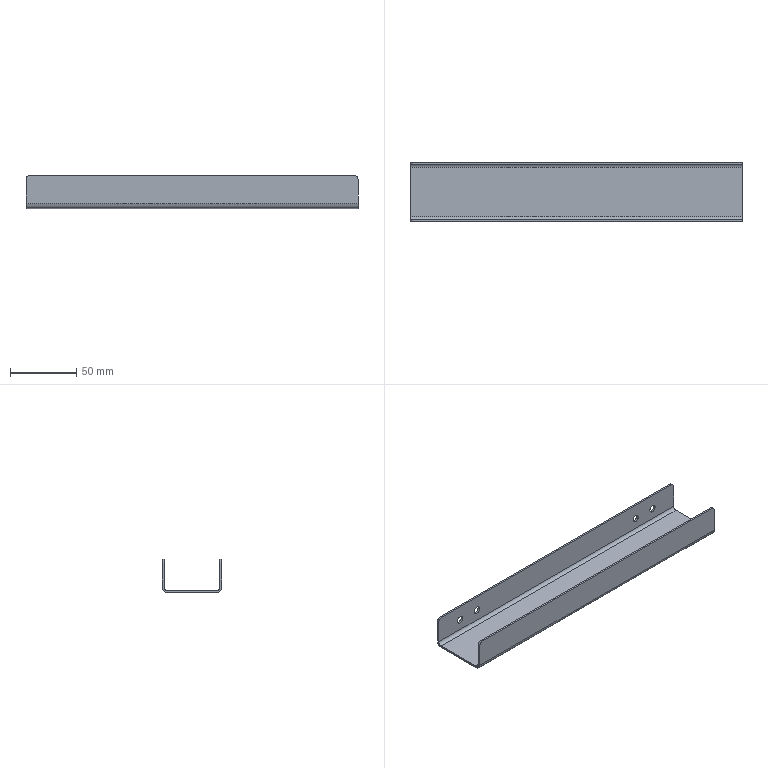Component | SolidWorks | FrameTransverseBeamOne40001100-1 | 1 solid | 34 faces | box 250 x 45 x 25 mm | volume 33300 mm3 | plane 18 | cylinder 16 | commonest cylinder face diameters 5.5 x8 6 x4 8 x2 5 x2
STEP:
#1=CARTESIAN_POINT('',(20.14,7.559,1.978));
#2=VERTEX_POINT('',#1);
#3=CARTESIAN_POINT('',(20.14,7.559,2.195));
#4=VERTEX_POINT('',#3);
#5=CARTESIAN_POINT('',(20.14,7.559,2.087));
#6=DIRECTION('',(-0.,1.,-0.));
#7=DIRECTION('',(0.,0.,-1.));
#8=AXIS2_PLACEMENT_3D('',#5,#6,#7);
#9=CIRCLE('',#8,0.1083);
#10=EDGE_CURVE('',#2,#4,#9,.T.);
#11=ORIENTED_EDGE('',*,*,#10,.F.);
#12=CARTESIAN_POINT('',(20.14,7.618,1.978));
#13=VERTEX_POINT('',#12);
#14=CARTESIAN_POINT('',(20.14,7.224,1.978));
#15=DIRECTION('',(-0.,1.,-0.));
#16=VECTOR('',#15,39.37);
#17=LINE('',#14,#16);
#18=EDGE_CURVE('',#2,#13,#17,.T.);
#19=ORIENTED_EDGE('',*,*,#18,.T.);
#20=CARTESIAN_POINT('',(20.14,7.618,2.195));
#21=VERTEX_POINT('',#20);
#22=CARTESIAN_POINT('',(20.14,7.618,2.087));
#23=DIRECTION('',(0.,-1.,0.));
#24=DIRECTION('',(0.,0.,1.));
#25=AXIS2_PLACEMENT_3D('',#22,#23,#24);
#26=CIRCLE('',#25,0.1083);
#27=EDGE_CURVE('',#21,#13,#26,.T.);
#28=ORIENTED_EDGE('',*,*,#27,.F.);
#29=CARTESIAN_POINT('',(20.14,7.224,2.195));
#30=DIRECTION('',(-0.,1.,-0.));
#31=VECTOR('',#30,39.37);
#32=LINE('',#29,#31);
#33=EDGE_CURVE('',#4,#21,#32,.T.);
#34=ORIENTED_EDGE('',*,*,#33,.F.);
#35=EDGE_LOOP('',(#11,#19,#28,#34));
#36=FACE_OUTER_BOUND('',#35,.T.);
#37=CARTESIAN_POINT('',(20.14,7.224,2.087));
#38=DIRECTION('',(-0.,1.,-0.));
#39=DIRECTION('',(0.,0.,1.));
#40=AXIS2_PLACEMENT_3D('',#37,#38,#39);
#41=CYLINDRICAL_SURFACE('',#40,0.1083);
#42=ADVANCED_FACE('',(#36),#41,.F.);
#43=CARTESIAN_POINT('',(20.849,7.559,1.978));
#44=VERTEX_POINT('',#43);
#45=CARTESIAN_POINT('',(20.849,7.559,2.195));
#46=VERTEX_POINT('',#45);
#47=CARTESIAN_POINT('',(20.849,7.559,2.087));
#48=DIRECTION('',(-0.,1.,-0.));
#49=DIRECTION('',(0.,0.,-1.));
#50=AXIS2_PLACEMENT_3D('',#47,#48,#49);
#51=CIRCLE('',#50,0.1083);
#52=EDGE_CURVE('',#44,#46,#51,.T.);
#53=ORIENTED_EDGE('',*,*,#52,.F.);
#54=CARTESIAN_POINT('',(20.849,7.618,1.978));
#55=VERTEX_POINT('',#54);
#56=CARTESIAN_POINT('',(20.849,7.224,1.978));
#57=DIRECTION('',(-0.,1.,-0.));
#58=VECTOR('',#57,39.37);
#59=LINE('',#56,#58);
#60=EDGE_CURVE('',#44,#55,#59,.T.);
#61=ORIENTED_EDGE('',*,*,#60,.T.);
#62=CARTESIAN_POINT('',(20.849,7.618,2.195));
#63=VERTEX_POINT('',#62);
#64=CARTESIAN_POINT('',(20.849,7.618,2.087));
#65=DIRECTION('',(0.,-1.,0.));
#66=DIRECTION('',(0.,0.,1.));
#67=AXIS2_PLACEMENT_3D('',#64,#65,#66);
#68=CIRCLE('',#67,0.1083);
#69=EDGE_CURVE('',#63,#55,#68,.T.);
#70=ORIENTED_EDGE('',*,*,#69,.F.);
#71=CARTESIAN_POINT('',(20.849,7.224,2.195));
#72=DIRECTION('',(-0.,1.,-0.));
#73=VECTOR('',#72,39.37);
#74=LINE('',#71,#73);
#75=EDGE_CURVE('',#46,#63,#74,.T.);
#76=ORIENTED_EDGE('',*,*,#75,.F.);
#77=EDGE_LOOP('',(#53,#61,#70,#76));
#78=FACE_OUTER_BOUND('',#77,.T.);
#79=CARTESIAN_POINT('',(20.849,7.224,2.087));
#80=DIRECTION('',(-0.,1.,-0.));
#81=DIRECTION('',(0.,0.,1.));
#82=AXIS2_PLACEMENT_3D('',#79,#80,#81);
#83=CYLINDRICAL_SURFACE('',#82,0.1083);
#84=ADVANCED_FACE('',(#78),#83,.F.);
#85=CARTESIAN_POINT('',(13.486,7.559,1.978));
#86=VERTEX_POINT('',#85);
#87=CARTESIAN_POINT('',(13.486,7.559,2.195));
#88=VERTEX_POINT('',#87);
#89=CARTESIAN_POINT('',(13.486,7.559,2.087));
#90=DIRECTION('',(-0.,1.,-0.));
#91=DIRECTION('',(0.,0.,-1.));
#92=AXIS2_PLACEMENT_3D('',#89,#90,#91);
#93=CIRCLE('',#92,0.1083);
#94=EDGE_CURVE('',#86,#88,#93,.T.);
#95=ORIENTED_EDGE('',*,*,#94,.F.);
#96=CARTESIAN_POINT('',(13.486,7.618,1.978));
#97=VERTEX_POINT('',#96);
#98=CARTESIAN_POINT('',(13.486,7.224,1.978));
#99=DIRECTION('',(-0.,1.,-0.));
#100=VECTOR('',#99,39.37);
#101=LINE('',#98,#100);
#102=EDGE_CURVE('',#86,#97,#101,.T.);
#103=ORIENTED_EDGE('',*,*,#102,.T.);
#104=CARTESIAN_POINT('',(13.486,7.618,2.195));
#105=VERTEX_POINT('',#104);
#106=CARTESIAN_POINT('',(13.486,7.618,2.087));
#107=DIRECTION('',(0.,-1.,0.));
#108=DIRECTION('',(0.,0.,-1.));
#109=AXIS2_PLACEMENT_3D('',#106,#107,#108);
#110=CIRCLE('',#109,0.1083);
#111=EDGE_CURVE('',#105,#97,#110,.T.);
#112=ORIENTED_EDGE('',*,*,#111,.F.);
#113=CARTESIAN_POINT('',(13.486,7.224,2.195));
#114=DIRECTION('',(-0.,1.,-0.));
#115=VECTOR('',#114,39.37);
#116=LINE('',#113,#115);
#117=EDGE_CURVE('',#88,#105,#116,.T.);
#118=ORIENTED_EDGE('',*,*,#117,.F.);
#119=EDGE_LOOP('',(#95,#103,#112,#118));
#120=FACE_OUTER_BOUND('',#119,.T.);
#121=CARTESIAN_POINT('',(13.486,7.224,2.087));
#122=DIRECTION('',(-0.,1.,-0.));
#123=DIRECTION('',(0.,0.,1.));
#124=AXIS2_PLACEMENT_3D('',#121,#122,#123);
#125=CYLINDRICAL_SURFACE('',#124,0.1083);
#126=ADVANCED_FACE('',(#120),#125,.F.);
#127=CARTESIAN_POINT('',(12.778,7.559,1.978));
#128=VERTEX_POINT('',#127);
#129=CARTESIAN_POINT('',(12.778,7.559,2.195));
#130=VERTEX_POINT('',#129);
#131=CARTESIAN_POINT('',(12.778,7.559,2.087));
#132=DIRECTION('',(-0.,1.,-0.));
#133=DIRECTION('',(0.,0.,-1.));
#134=AXIS2_PLACEMENT_3D('',#131,#132,#133);
#135=CIRCLE('',#134,0.1083);
#136=EDGE_CURVE('',#128,#130,#135,.T.);
#137=ORIENTED_EDGE('',*,*,#136,.F.);
#138=CARTESIAN_POINT('',(12.778,7.618,1.978));
#139=VERTEX_POINT('',#138);
#140=CARTESIAN_POINT('',(12.778,7.224,1.978));
#141=DIRECTION('',(-0.,1.,-0.));
#142=VECTOR('',#141,39.37);
#143=LINE('',#140,#142);
#144=EDGE_CURVE('',#128,#139,#143,.T.);
#145=ORIENTED_EDGE('',*,*,#144,.T.);
#146=CARTESIAN_POINT('',(12.778,7.618,2.195));
#147=VERTEX_POINT('',#146);
#148=CARTESIAN_POINT('',(12.778,7.618,2.087));
#149=DIRECTION('',(0.,-1.,0.));
#150=DIRECTION('',(0.,0.,-1.));
#151=AXIS2_PLACEMENT_3D('',#148,#149,#150);
#152=CIRCLE('',#151,0.1083);
#153=EDGE_CURVE('',#147,#139,#152,.T.);
#154=ORIENTED_EDGE('',*,*,#153,.F.);
#155=CARTESIAN_POINT('',(12.778,7.224,2.195));
#156=DIRECTION('',(-0.,1.,-0.));
#157=VECTOR('',#156,39.37);
#158=LINE('',#155,#157);
#159=EDGE_CURVE('',#130,#147,#158,.T.);
#160=ORIENTED_EDGE('',*,*,#159,.F.);
#161=EDGE_LOOP('',(#137,#145,#154,#160));
#162=FACE_OUTER_BOUND('',#161,.T.);
#163=CARTESIAN_POINT('',(12.778,7.224,2.087));
#164=DIRECTION('',(-0.,1.,-0.));
#165=DIRECTION('',(0.,0.,1.));
#166=AXIS2_PLACEMENT_3D('',#163,#164,#165);
#167=CYLINDRICAL_SURFACE('',#166,0.1083);
#168=ADVANCED_FACE('',(#162),#167,.F.);
#169=ORIENTED_EDGE('',*,*,#69,.T.);
#170=CARTESIAN_POINT('',(20.849,7.618,2.087));
#171=DIRECTION('',(0.,-1.,0.));
#172=DIRECTION('',(0.,0.,1.));
#173=AXIS2_PLACEMENT_3D('',#170,#171,#172);
#174=CIRCLE('',#173,0.1083);
#175=EDGE_CURVE('',#55,#63,#174,.T.);
#176=ORIENTED_EDGE('',*,*,#175,.T.);
#177=EDGE_LOOP('',(#169,#176));
#178=FACE_BOUND('',#177,.T.);
#179=ORIENTED_EDGE('',*,*,#153,.T.);
#180=CARTESIAN_POINT('',(12.778,7.618,2.087));
#181=DIRECTION('',(0.,-1.,0.));
#182=DIRECTION('',(0.,0.,-1.));
#183=AXIS2_PLACEMENT_3D('',#180,#181,#182);
#184=CIRCLE('',#183,0.1083);
#185=EDGE_CURVE('',#139,#147,#184,.T.);
#186=ORIENTED_EDGE('',*,*,#185,.T.);
#187=EDGE_LOOP('',(#179,#186));
#188=FACE_BOUND('',#187,.T.);
#189=CARTESIAN_POINT('',(12.01,7.618,2.559));
#190=VERTEX_POINT('',#189);
#191=CARTESIAN_POINT('',(21.616,7.618,2.559));
#192=VERTEX_POINT('',#191);
#193=CARTESIAN_POINT('',(21.734,7.618,2.559));
#194=DIRECTION('',(1.,0.,0.));
#195=VECTOR('',#194,39.37);
#196=LINE('',#193,#195);
#197=EDGE_CURVE('',#190,#192,#196,.T.);
#198=ORIENTED_EDGE('',*,*,#197,.T.);
#199=CARTESIAN_POINT('',(21.734,7.618,2.441));
#200=VERTEX_POINT('',#199);
#201=CARTESIAN_POINT('',(21.616,7.618,2.441));
#202=DIRECTION('',(-0.,1.,-0.));
#203=DIRECTION('',(0.,0.,-1.));
#204=AXIS2_PLACEMENT_3D('',#201,#202,#203);
#205=CIRCLE('',#204,0.1181);
#206=EDGE_CURVE('',#192,#200,#205,.T.);
#207=ORIENTED_EDGE('',*,*,#206,.T.);
#208=CARTESIAN_POINT('',(21.734,7.618,1.732));
#209=VERTEX_POINT('',#208);
#210=CARTESIAN_POINT('',(21.734,7.618,2.559));
#211=DIRECTION('',(-0.,-0.,-1.));
#212=VECTOR('',#211,39.37);
#213=LINE('',#210,#212);
#214=EDGE_CURVE('',#200,#209,#213,.T.);
#215=ORIENTED_EDGE('',*,*,#214,.T.);
#216=CARTESIAN_POINT('',(11.892,7.618,1.732));
#217=VERTEX_POINT('',#216);
#218=CARTESIAN_POINT('',(21.734,7.618,1.732));
#219=DIRECTION('',(1.,0.,0.));
#220=VECTOR('',#219,39.37);
#221=LINE('',#218,#220);
#222=EDGE_CURVE('',#217,#209,#221,.T.);
#223=ORIENTED_EDGE('',*,*,#222,.F.);
#224=CARTESIAN_POINT('',(11.892,7.618,2.441));
#225=VERTEX_POINT('',#224);
#226=CARTESIAN_POINT('',(11.892,7.618,2.559));
#227=DIRECTION('',(-0.,0.,1.));
#228=VECTOR('',#227,39.37);
#229=LINE('',#226,#228);
#230=EDGE_CURVE('',#217,#225,#229,.T.);
#231=ORIENTED_EDGE('',*,*,#230,.T.);
#232=CARTESIAN_POINT('',(12.01,7.618,2.441));
#233=DIRECTION('',(-0.,1.,-0.));
#234=DIRECTION('',(0.,0.,-1.));
#235=AXIS2_PLACEMENT_3D('',#232,#233,#234);
#236=CIRCLE('',#235,0.1181);
#237=EDGE_CURVE('',#225,#190,#236,.T.);
#238=ORIENTED_EDGE('',*,*,#237,.T.);
#239=EDGE_LOOP('',(#198,#207,#215,#223,#231,#238));
#240=FACE_OUTER_BOUND('',#239,.T.);
#241=ORIENTED_EDGE('',*,*,#111,.T.);
#242=CARTESIAN_POINT('',(13.486,7.618,2.087));
#243=DIRECTION('',(0.,-1.,0.));
#244=DIRECTION('',(0.,0.,-1.));
#245=AXIS2_PLACEMENT_3D('',#242,#243,#244);
#246=CIRCLE('',#245,0.1083);
#247=EDGE_CURVE('',#97,#105,#246,.T.);
#248=ORIENTED_EDGE('',*,*,#247,.T.);
#249=EDGE_LOOP('',(#241,#248));
#250=FACE_BOUND('',#249,.T.);
#251=ORIENTED_EDGE('',*,*,#27,.T.);
#252=CARTESIAN_POINT('',(20.14,7.618,2.087));
#253=DIRECTION('',(0.,-1.,0.));
#254=DIRECTION('',(0.,0.,1.));
#255=AXIS2_PLACEMENT_3D('',#252,#253,#254);
#256=CIRCLE('',#255,0.1083);
#257=EDGE_CURVE('',#13,#21,#256,.T.);
#258=ORIENTED_EDGE('',*,*,#257,.T.);
#259=EDGE_LOOP('',(#251,#258));
#260=FACE_BOUND('',#259,.T.);
#261=CARTESIAN_POINT('',(21.734,7.618,2.559));
#262=DIRECTION('',(0.,-1.,0.));
#263=DIRECTION('',(0.,-0.,-1.));
#264=AXIS2_PLACEMENT_3D('',#261,#262,#263);
#265=PLANE('',#264);
#266=ADVANCED_FACE('',(#178,#188,#240,#250,#260),#265,.F.);
#267=CARTESIAN_POINT('',(20.849,7.559,2.087));
#268=DIRECTION('',(-0.,1.,-0.));
#269=DIRECTION('',(0.,0.,-1.));
#270=AXIS2_PLACEMENT_3D('',#267,#268,#269);
#271=CIRCLE('',#270,0.1083);
#272=EDGE_CURVE('',#46,#44,#271,.T.);
#273=ORIENTED_EDGE('',*,*,#272,.T.);
#274=ORIENTED_EDGE('',*,*,#52,.T.);
#275=EDGE_LOOP('',(#273,#274));
#276=FACE_BOUND('',#275,.T.);
#277=CARTESIAN_POINT('',(12.778,7.559,2.087));
#278=DIRECTION('',(-0.,1.,-0.));
#279=DIRECTION('',(0.,0.,-1.));
#280=AXIS2_PLACEMENT_3D('',#277,#278,#279);
#281=CIRCLE('',#280,0.1083);
#282=EDGE_CURVE('',#130,#128,#281,.T.);
#283=ORIENTED_EDGE('',*,*,#282,.T.);
#284=ORIENTED_EDGE('',*,*,#136,.T.);
#285=EDGE_LOOP('',(#283,#284));
#286=FACE_BOUND('',#285,.T.);
#287=CARTESIAN_POINT('',(21.734,7.559,2.441));
#288=VERTEX_POINT('',#287);
#289=CARTESIAN_POINT('',(21.734,7.559,1.732));
#290=VERTEX_POINT('',#289);
#291=CARTESIAN_POINT('',(21.734,7.559,1.634));
#292=DIRECTION('',(-0.,-0.,-1.));
#293=VECTOR('',#292,39.37);
#294=LINE('',#291,#293);
#295=EDGE_CURVE('',#288,#290,#294,.T.);
#296=ORIENTED_EDGE('',*,*,#295,.F.);
#297=CARTESIAN_POINT('',(21.616,7.559,2.559));
#298=VERTEX_POINT('',#297);
#299=CARTESIAN_POINT('',(21.616,7.559,2.441));
#300=DIRECTION('',(0.,-1.,0.));
#301=DIRECTION('',(0.,0.,-1.));
#302=AXIS2_PLACEMENT_3D('',#299,#300,#301);
#303=CIRCLE('',#302,0.1181);
#304=EDGE_CURVE('',#288,#298,#303,.T.);
#305=ORIENTED_EDGE('',*,*,#304,.T.);
#306=CARTESIAN_POINT('',(12.01,7.559,2.559));
#307=VERTEX_POINT('',#306);
#308=CARTESIAN_POINT('',(21.734,7.559,2.559));
#309=DIRECTION('',(1.,0.,0.));
#310=VECTOR('',#309,39.37);
#311=LINE('',#308,#310);
#312=EDGE_CURVE('',#307,#298,#311,.T.);
#313=ORIENTED_EDGE('',*,*,#312,.F.);
#314=CARTESIAN_POINT('',(11.892,7.559,2.441));
#315=VERTEX_POINT('',#314);
#316=CARTESIAN_POINT('',(12.01,7.559,2.441));
#317=DIRECTION('',(0.,-1.,0.));
#318=DIRECTION('',(0.,0.,-1.));
#319=AXIS2_PLACEMENT_3D('',#316,#317,#318);
#320=CIRCLE('',#319,0.1181);
#321=EDGE_CURVE('',#307,#315,#320,.T.);
#322=ORIENTED_EDGE('',*,*,#321,.T.);
#323=CARTESIAN_POINT('',(11.892,7.559,1.732));
#324=VERTEX_POINT('',#323);
#325=CARTESIAN_POINT('',(11.892,7.559,2.559));
#326=DIRECTION('',(-0.,0.,1.));
#327=VECTOR('',#326,39.37);
#328=LINE('',#325,#327);
#329=EDGE_CURVE('',#324,#315,#328,.T.);
#330=ORIENTED_EDGE('',*,*,#329,.F.);
#331=CARTESIAN_POINT('',(21.734,7.559,1.732));
#332=DIRECTION('',(-1.,-0.,0.));
#333=VECTOR('',#332,39.37);
#334=LINE('',#331,#333);
#335=EDGE_CURVE('',#290,#324,#334,.T.);
#336=ORIENTED_EDGE('',*,*,#335,.F.);
#337=EDGE_LOOP('',(#296,#305,#313,#322,#330,#336));
#338=FACE_OUTER_BOUND('',#337,.T.);
#339=CARTESIAN_POINT('',(13.486,7.559,2.087));
#340=DIRECTION('',(-0.,1.,-0.));
#341=DIRECTION('',(0.,0.,-1.));
#342=AXIS2_PLACEMENT_3D('',#339,#340,#341);
#343=CIRCLE('',#342,0.1083);
#344=EDGE_CURVE('',#88,#86,#343,.T.);
#345=ORIENTED_EDGE('',*,*,#344,.T.);
#346=ORIENTED_EDGE('',*,*,#94,.T.);
#347=EDGE_LOOP('',(#345,#346));
#348=FACE_BOUND('',#347,.T.);
#349=CARTESIAN_POINT('',(20.14,7.559,2.087));
#350=DIRECTION('',(-0.,1.,-0.));
#351=DIRECTION('',(0.,0.,-1.));
#352=AXIS2_PLACEMENT_3D('',#349,#350,#351);
#353=CIRCLE('',#352,0.1083);
#354=EDGE_CURVE('',#4,#2,#353,.T.);
#355=ORIENTED_EDGE('',*,*,#354,.T.);
#356=ORIENTED_EDGE('',*,*,#10,.T.);
#357=EDGE_LOOP('',(#355,#356));
#358=FACE_BOUND('',#357,.T.);
#359=CARTESIAN_POINT('',(21.734,7.559,2.559));
#360=DIRECTION('',(0.,-1.,0.));
#361=DIRECTION('',(0.,-0.,-1.));
#362=AXIS2_PLACEMENT_3D('',#359,#360,#361);
#363=PLANE('',#362);
#364=ADVANCED_FACE('',(#276,#286,#338,#348,#358),#363,.T.);
#365=CARTESIAN_POINT('',(21.734,6.004,1.575));
#366=VERTEX_POINT('',#365);
#367=CARTESIAN_POINT('',(11.892,6.004,1.575));
#368=VERTEX_POINT('',#367);
#369=CARTESIAN_POINT('',(21.734,6.004,1.575));
#370=DIRECTION('',(-1.,-0.,0.));
#371=VECTOR('',#370,39.37);
#372=LINE('',#369,#371);
#373=EDGE_CURVE('',#366,#368,#372,.T.);
#374=ORIENTED_EDGE('',*,*,#373,.T.);
#375=CARTESIAN_POINT('',(11.892,7.461,1.575));
#376=VERTEX_POINT('',#375);
#377=CARTESIAN_POINT('',(11.892,5.846,1.575));
#378=DIRECTION('',(0.,-1.,0.));
#379=VECTOR('',#378,39.37);
#380=LINE('',#377,#379);
#381=EDGE_CURVE('',#376,#368,#380,.T.);
#382=ORIENTED_EDGE('',*,*,#381,.F.);
#383=CARTESIAN_POINT('',(21.734,7.461,1.575));
#384=VERTEX_POINT('',#383);
#385=CARTESIAN_POINT('',(11.892,7.461,1.575));
#386=DIRECTION('',(1.,0.,0.));
#387=VECTOR('',#386,39.37);
#388=LINE('',#385,#387);
#389=EDGE_CURVE('',#376,#384,#388,.T.);
#390=ORIENTED_EDGE('',*,*,#389,.T.);
#391=CARTESIAN_POINT('',(21.734,5.846,1.575));
#392=DIRECTION('',(0.,1.,0.));
#393=VECTOR('',#392,39.37);
#394=LINE('',#391,#393);
#395=EDGE_CURVE('',#366,#384,#394,.T.);
#396=ORIENTED_EDGE('',*,*,#395,.F.);
#397=EDGE_LOOP('',(#374,#382,#390,#396));
#398=FACE_OUTER_BOUND('',#397,.T.);
#399=CARTESIAN_POINT('',(21.734,7.618,1.575));
#400=DIRECTION('',(0.,0.,1.));
#401=DIRECTION('',(1.,0.,0.));
#402=AXIS2_PLACEMENT_3D('',#399,#400,#401);
#403=PLANE('',#402);
#404=ADVANCED_FACE('',(#398),#403,.F.);
#405=CARTESIAN_POINT('',(11.892,7.461,1.634));
#406=VERTEX_POINT('',#405);
#407=CARTESIAN_POINT('',(11.892,6.004,1.634));
#408=VERTEX_POINT('',#407);
#409=CARTESIAN_POINT('',(11.892,5.846,1.634));
#410=DIRECTION('',(0.,-1.,0.));
#411=VECTOR('',#410,39.37);
#412=LINE('',#409,#411);
#413=EDGE_CURVE('',#406,#408,#412,.T.);
#414=ORIENTED_EDGE('',*,*,#413,.T.);
#415=CARTESIAN_POINT('',(21.734,6.004,1.634));
#416=VERTEX_POINT('',#415);
#417=CARTESIAN_POINT('',(21.734,6.004,1.634));
#418=DIRECTION('',(-1.,-0.,0.));
#419=VECTOR('',#418,39.37);
#420=LINE('',#417,#419);
#421=EDGE_CURVE('',#416,#408,#420,.T.);
#422=ORIENTED_EDGE('',*,*,#421,.F.);
#423=CARTESIAN_POINT('',(21.734,7.461,1.634));
#424=VERTEX_POINT('',#423);
#425=CARTESIAN_POINT('',(21.734,5.846,1.634));
#426=DIRECTION('',(0.,1.,0.));
#427=VECTOR('',#426,39.37);
#428=LINE('',#425,#427);
#429=EDGE_CURVE('',#416,#424,#428,.T.);
#430=ORIENTED_EDGE('',*,*,#429,.T.);
#431=CARTESIAN_POINT('',(11.892,7.461,1.634));
#432=DIRECTION('',(1.,0.,0.));
#433=VECTOR('',#432,39.37);
#434=LINE('',#431,#433);
#435=EDGE_CURVE('',#406,#424,#434,.T.);
#436=ORIENTED_EDGE('',*,*,#435,.F.);
#437=EDGE_LOOP('',(#414,#422,#430,#436));
#438=FACE_OUTER_BOUND('',#437,.T.);
#439=CARTESIAN_POINT('',(21.734,7.618,1.634));
#440=DIRECTION('',(0.,0.,1.));
#441=DIRECTION('',(1.,0.,0.));
#442=AXIS2_PLACEMENT_3D('',#439,#440,#441);
#443=PLANE('',#442);
#444=ADVANCED_FACE('',(#438),#443,.T.);
#445=ORIENTED_EDGE('',*,*,#429,.F.);
#446=CARTESIAN_POINT('',(21.734,6.004,1.634));
#447=DIRECTION('',(0.,-0.,-1.));
#448=VECTOR('',#447,39.37);
#449=LINE('',#446,#448);
#450=EDGE_CURVE('',#416,#366,#449,.T.);
#451=ORIENTED_EDGE('',*,*,#450,.T.);
#452=ORIENTED_EDGE('',*,*,#395,.T.);
#453=CARTESIAN_POINT('',(21.734,7.461,1.634));
#454=DIRECTION('',(0.,-0.,-1.));
#455=VECTOR('',#454,39.37);
#456=LINE('',#453,#455);
#457=EDGE_CURVE('',#424,#384,#456,.T.);
#458=ORIENTED_EDGE('',*,*,#457,.F.);
#459=EDGE_LOOP('',(#445,#451,#452,#458));
#460=FACE_OUTER_BOUND('',#459,.T.);
#461=CARTESIAN_POINT('',(21.734,5.846,1.575));
#462=DIRECTION('',(1.,0.,0.));
#463=DIRECTION('',(0.,0.,-1.));
#464=AXIS2_PLACEMENT_3D('',#461,#462,#463);
#465=PLANE('',#464);
#466=ADVANCED_FACE('',(#460),#465,.T.);
#467=CARTESIAN_POINT('',(11.892,6.004,1.634));
#468=DIRECTION('',(0.,-0.,-1.));
#469=VECTOR('',#468,39.37);
#470=LINE('',#467,#469);
#471=EDGE_CURVE('',#408,#368,#470,.T.);
#472=ORIENTED_EDGE('',*,*,#471,.F.);
#473=ORIENTED_EDGE('',*,*,#413,.F.);
#474=CARTESIAN_POINT('',(11.892,7.461,1.634));
#475=DIRECTION('',(0.,-0.,-1.));
#476=VECTOR('',#475,39.37);
#477=LINE('',#474,#476);
#478=EDGE_CURVE('',#406,#376,#477,.T.);
#479=ORIENTED_EDGE('',*,*,#478,.T.);
#480=ORIENTED_EDGE('',*,*,#381,.T.);
#481=EDGE_LOOP('',(#472,#473,#479,#480));
#482=FACE_OUTER_BOUND('',#481,.T.);
#483=CARTESIAN_POINT('',(11.892,5.846,1.575));
#484=DIRECTION('',(-1.,0.,0.));
#485=DIRECTION('',(0.,0.,1.));
#486=AXIS2_PLACEMENT_3D('',#483,#484,#485);
#487=PLANE('',#486);
#488=ADVANCED_FACE('',(#482),#487,.T.);
#489=CARTESIAN_POINT('',(21.734,7.618,1.732));
#490=DIRECTION('',(-0.,1.,-0.));
#491=VECTOR('',#490,39.37);
#492=LINE('',#489,#491);
#493=EDGE_CURVE('',#290,#209,#492,.T.);
#494=ORIENTED_EDGE('',*,*,#493,.F.);
#495=CARTESIAN_POINT('',(21.734,7.461,1.732));
#496=DIRECTION('',(1.,0.,0.));
#497=DIRECTION('',(0.,0.,1.));
#498=AXIS2_PLACEMENT_3D('',#495,#496,#497);
#499=CIRCLE('',#498,0.09843);
#500=EDGE_CURVE('',#424,#290,#499,.T.);
#501=ORIENTED_EDGE('',*,*,#500,.F.);
#502=ORIENTED_EDGE('',*,*,#457,.T.);
#503=CARTESIAN_POINT('',(21.734,7.461,1.732));
#504=DIRECTION('',(1.,0.,0.));
#505=DIRECTION('',(0.,0.,1.));
#506=AXIS2_PLACEMENT_3D('',#503,#504,#505);
#507=CIRCLE('',#506,0.1575);
#508=EDGE_CURVE('',#384,#209,#507,.T.);
#509=ORIENTED_EDGE('',*,*,#508,.T.);
#510=EDGE_LOOP('',(#494,#501,#502,#509));
#511=FACE_OUTER_BOUND('',#510,.T.);
#512=CARTESIAN_POINT('',(21.734,7.461,1.732));
#513=DIRECTION('',(1.,0.,0.));
#514=DIRECTION('',(0.,0.,-1.));
#515=AXIS2_PLACEMENT_3D('',#512,#513,#514);
#516=PLANE('',#515);
#517=ADVANCED_FACE('',(#511),#516,.T.);
#518=ORIENTED_EDGE('',*,*,#389,.F.);
#519=CARTESIAN_POINT('',(11.892,7.461,1.732));
#520=DIRECTION('',(-1.,0.,0.));
#521=DIRECTION('',(0.,0.,1.));
#522=AXIS2_PLACEMENT_3D('',#519,#520,#521);
#523=CIRCLE('',#522,0.1575);
#524=EDGE_CURVE('',#217,#376,#523,.T.);
#525=ORIENTED_EDGE('',*,*,#524,.F.);
#526=ORIENTED_EDGE('',*,*,#222,.T.);
#527=ORIENTED_EDGE('',*,*,#508,.F.);
#528=EDGE_LOOP('',(#518,#525,#526,#527));
#529=FACE_OUTER_BOUND('',#528,.T.);
#530=CARTESIAN_POINT('',(11.892,7.461,1.732));
#531=DIRECTION('',(-1.,0.,0.));
#532=DIRECTION('',(0.,1.,-0.));
#533=AXIS2_PLACEMENT_3D('',#530,#531,#532);
#534=CYLINDRICAL_SURFACE('',#533,0.1575);
#535=ADVANCED_FACE('',(#529),#534,.T.);
#536=CARTESIAN_POINT('',(11.892,7.461,1.732));
#537=DIRECTION('',(-1.,0.,0.));
#538=DIRECTION('',(0.,0.,1.));
#539=AXIS2_PLACEMENT_3D('',#536,#537,#538);
#540=CIRCLE('',#539,0.09843);
#541=EDGE_CURVE('',#324,#406,#540,.T.);
#542=ORIENTED_EDGE('',*,*,#541,.F.);
#543=CARTESIAN_POINT('',(11.892,7.559,1.732));
#544=DIRECTION('',(-0.,1.,-0.));
#545=VECTOR('',#544,39.37);
#546=LINE('',#543,#545);
#547=EDGE_CURVE('',#324,#217,#546,.T.);
#548=ORIENTED_EDGE('',*,*,#547,.T.);
#549=ORIENTED_EDGE('',*,*,#524,.T.);
#550=ORIENTED_EDGE('',*,*,#478,.F.);
#551=EDGE_LOOP('',(#542,#548,#549,#550));
#552=FACE_OUTER_BOUND('',#551,.T.);
#553=CARTESIAN_POINT('',(11.892,7.461,1.732));
#554=DIRECTION('',(1.,0.,0.));
#555=DIRECTION('',(0.,0.,-1.));
#556=AXIS2_PLACEMENT_3D('',#553,#554,#555);
#557=PLANE('',#556);
#558=ADVANCED_FACE('',(#552),#557,.F.);
#559=ORIENTED_EDGE('',*,*,#435,.T.);
#560=ORIENTED_EDGE('',*,*,#500,.T.);
#561=ORIENTED_EDGE('',*,*,#335,.T.);
#562=ORIENTED_EDGE('',*,*,#541,.T.);
#563=EDGE_LOOP('',(#559,#560,#561,#562));
#564=FACE_OUTER_BOUND('',#563,.T.);
#565=CARTESIAN_POINT('',(11.892,7.461,1.732));
#566=DIRECTION('',(-1.,0.,0.));
#567=DIRECTION('',(0.,1.,-0.));
#568=AXIS2_PLACEMENT_3D('',#565,#566,#567);
#569=CYLINDRICAL_SURFACE('',#568,0.09843);
#570=ADVANCED_FACE('',(#564),#569,.F.);
#571=ORIENTED_EDGE('',*,*,#214,.F.);
#572=CARTESIAN_POINT('',(21.734,7.618,2.441));
#573=DIRECTION('',(0.,-1.,0.));
#574=VECTOR('',#573,39.37);
#575=LINE('',#572,#574);
#576=EDGE_CURVE('',#200,#288,#575,.T.);
#577=ORIENTED_EDGE('',*,*,#576,.T.);
#578=ORIENTED_EDGE('',*,*,#295,.T.);
#579=ORIENTED_EDGE('',*,*,#493,.T.);
#580=EDGE_LOOP('',(#571,#577,#578,#579));
#581=FACE_OUTER_BOUND('',#580,.T.);
#582=CARTESIAN_POINT('',(21.734,7.618,1.634));
#583=DIRECTION('',(-1.,-0.,0.));
#584=DIRECTION('',(0.,-1.,0.));
#585=AXIS2_PLACEMENT_3D('',#582,#583,#584);
#586=PLANE('',#585);
#587=ADVANCED_FACE('',(#581),#586,.F.);
#588=ORIENTED_EDGE('',*,*,#329,.T.);
#589=CARTESIAN_POINT('',(11.892,7.618,2.441));
#590=DIRECTION('',(-0.,1.,-0.));
#591=VECTOR('',#590,39.37);
#592=LINE('',#589,#591);
#593=EDGE_CURVE('',#315,#225,#592,.T.);
#594=ORIENTED_EDGE('',*,*,#593,.T.);
#595=ORIENTED_EDGE('',*,*,#230,.F.);
#596=ORIENTED_EDGE('',*,*,#547,.F.);
#597=EDGE_LOOP('',(#588,#594,#595,#596));
#598=FACE_OUTER_BOUND('',#597,.T.);
#599=CARTESIAN_POINT('',(11.892,7.618,2.559));
#600=DIRECTION('',(1.,0.,-0.));
#601=DIRECTION('',(-0.,1.,0.));
#602=AXIS2_PLACEMENT_3D('',#599,#600,#601);
#603=PLANE('',#602);
#604=ADVANCED_FACE('',(#598),#603,.F.);
#605=ORIENTED_EDGE('',*,*,#312,.T.);
#606=CARTESIAN_POINT('',(21.616,7.618,2.559));
#607=DIRECTION('',(-0.,1.,-0.));
#608=VECTOR('',#607,39.37);
#609=LINE('',#606,#608);
#610=EDGE_CURVE('',#298,#192,#609,.T.);
#611=ORIENTED_EDGE('',*,*,#610,.T.);
#612=ORIENTED_EDGE('',*,*,#197,.F.);
#613=CARTESIAN_POINT('',(12.01,7.618,2.559));
#614=DIRECTION('',(0.,-1.,0.));
#615=VECTOR('',#614,39.37);
#616=LINE('',#613,#615);
#617=EDGE_CURVE('',#190,#307,#616,.T.);
#618=ORIENTED_EDGE('',*,*,#617,.T.);
#619=EDGE_LOOP('',(#605,#611,#612,#618));
#620=FACE_OUTER_BOUND('',#619,.T.);
#621=CARTESIAN_POINT('',(21.734,7.618,2.559));
#622=DIRECTION('',(0.,-0.,-1.));
#623=DIRECTION('',(0.,1.,-0.));
#624=AXIS2_PLACEMENT_3D('',#621,#622,#623);
#625=PLANE('',#624);
#626=ADVANCED_FACE('',(#620),#625,.F.);
#627=CARTESIAN_POINT('',(11.892,5.905,1.732));
#628=VERTEX_POINT('',#627);
#629=CARTESIAN_POINT('',(11.892,5.846,1.732));
#630=VERTEX_POINT('',#629);
#631=CARTESIAN_POINT('',(11.892,5.846,1.732));
#632=DIRECTION('',(0.,-1.,-0.));
#633=VECTOR('',#632,39.37);
#634=LINE('',#631,#633);
#635=EDGE_CURVE('',#628,#630,#634,.T.);
#636=ORIENTED_EDGE('',*,*,#635,.F.);
#637=CARTESIAN_POINT('',(11.892,6.004,1.732));
#638=DIRECTION('',(-1.,-0.,0.));
#639=DIRECTION('',(0.,1.,0.));
#640=AXIS2_PLACEMENT_3D('',#637,#638,#639);
#641=CIRCLE('',#640,0.09843);
#642=EDGE_CURVE('',#408,#628,#641,.T.);
#643=ORIENTED_EDGE('',*,*,#642,.F.);
#644=ORIENTED_EDGE('',*,*,#471,.T.);
#645=CARTESIAN_POINT('',(11.892,6.004,1.732));
#646=DIRECTION('',(-1.,-0.,0.));
#647=DIRECTION('',(0.,1.,0.));
#648=AXIS2_PLACEMENT_3D('',#645,#646,#647);
#649=CIRCLE('',#648,0.1575);
#650=EDGE_CURVE('',#368,#630,#649,.T.);
#651=ORIENTED_EDGE('',*,*,#650,.T.);
#652=EDGE_LOOP('',(#636,#643,#644,#651));
#653=FACE_OUTER_BOUND('',#652,.T.);
#654=CARTESIAN_POINT('',(11.892,6.004,1.732));
#655=DIRECTION('',(-1.,-0.,0.));
#656=DIRECTION('',(0.,-1.,0.));
#657=AXIS2_PLACEMENT_3D('',#654,#655,#656);
#658=PLANE('',#657);
#659=ADVANCED_FACE('',(#653),#658,.T.);
#660=ORIENTED_EDGE('',*,*,#373,.F.);
#661=CARTESIAN_POINT('',(21.734,5.846,1.732));
#662=VERTEX_POINT('',#661);
#663=CARTESIAN_POINT('',(21.734,6.004,1.732));
#664=DIRECTION('',(1.,0.,0.));
#665=DIRECTION('',(0.,1.,0.));
#666=AXIS2_PLACEMENT_3D('',#663,#664,#665);
#667=CIRCLE('',#666,0.1575);
#668=EDGE_CURVE('',#662,#366,#667,.T.);
#669=ORIENTED_EDGE('',*,*,#668,.F.);
#670=CARTESIAN_POINT('',(11.892,5.846,1.732));
#671=DIRECTION('',(-1.,-0.,-0.));
#672=VECTOR('',#671,39.37);
#673=LINE('',#670,#672);
#674=EDGE_CURVE('',#662,#630,#673,.T.);
#675=ORIENTED_EDGE('',*,*,#674,.T.);
#676=ORIENTED_EDGE('',*,*,#650,.F.);
#677=EDGE_LOOP('',(#660,#669,#675,#676));
#678=FACE_OUTER_BOUND('',#677,.T.);
#679=CARTESIAN_POINT('',(21.734,6.004,1.732));
#680=DIRECTION('',(1.,0.,0.));
#681=DIRECTION('',(0.,-1.,-0.));
#682=AXIS2_PLACEMENT_3D('',#679,#680,#681);
#683=CYLINDRICAL_SURFACE('',#682,0.1575);
#684=ADVANCED_FACE('',(#678),#683,.T.);
#685=CARTESIAN_POINT('',(21.734,5.905,1.732));
#686=VERTEX_POINT('',#685);
#687=CARTESIAN_POINT('',(21.734,6.004,1.732));
#688=DIRECTION('',(1.,0.,0.));
#689=DIRECTION('',(0.,1.,0.));
#690=AXIS2_PLACEMENT_3D('',#687,#688,#689);
#691=CIRCLE('',#690,0.09843);
#692=EDGE_CURVE('',#686,#416,#691,.T.);
#693=ORIENTED_EDGE('',*,*,#692,.F.);
#694=CARTESIAN_POINT('',(21.734,5.905,1.732));
#695=DIRECTION('',(0.,-1.,-0.));
#696=VECTOR('',#695,39.37);
#697=LINE('',#694,#696);
#698=EDGE_CURVE('',#686,#662,#697,.T.);
#699=ORIENTED_EDGE('',*,*,#698,.T.);
#700=ORIENTED_EDGE('',*,*,#668,.T.);
#701=ORIENTED_EDGE('',*,*,#450,.F.);
#702=EDGE_LOOP('',(#693,#699,#700,#701));
#703=FACE_OUTER_BOUND('',#702,.T.);
#704=CARTESIAN_POINT('',(21.734,6.004,1.732));
#705=DIRECTION('',(-1.,-0.,0.));
#706=DIRECTION('',(0.,-1.,0.));
#707=AXIS2_PLACEMENT_3D('',#704,#705,#706);
#708=PLANE('',#707);
#709=ADVANCED_FACE('',(#703),#708,.F.);
#710=ORIENTED_EDGE('',*,*,#421,.T.);
#711=ORIENTED_EDGE('',*,*,#642,.T.);
#712=CARTESIAN_POINT('',(11.892,5.905,1.732));
#713=DIRECTION('',(1.,0.,0.));
#714=VECTOR('',#713,39.37);
#715=LINE('',#712,#714);
#716=EDGE_CURVE('',#628,#686,#715,.T.);
#717=ORIENTED_EDGE('',*,*,#716,.T.);
#718=ORIENTED_EDGE('',*,*,#692,.T.);
#719=EDGE_LOOP('',(#710,#711,#717,#718));
#720=FACE_OUTER_BOUND('',#719,.T.);
#721=CARTESIAN_POINT('',(21.734,6.004,1.732));
#722=DIRECTION('',(1.,0.,0.));
#723=DIRECTION('',(0.,-1.,-0.));
#724=AXIS2_PLACEMENT_3D('',#721,#722,#723);
#725=CYLINDRICAL_SURFACE('',#724,0.09843);
#726=ADVANCED_FACE('',(#720),#725,.F.);
#727=CARTESIAN_POINT('',(11.892,5.846,2.441));
#728=VERTEX_POINT('',#727);
#729=CARTESIAN_POINT('',(11.892,5.846,2.559));
#730=DIRECTION('',(0.,0.,-1.));
#731=VECTOR('',#730,39.37);
#732=LINE('',#729,#731);
#733=EDGE_CURVE('',#728,#630,#732,.T.);
#734=ORIENTED_EDGE('',*,*,#733,.F.);
#735=CARTESIAN_POINT('',(11.892,5.905,2.441));
#736=VERTEX_POINT('',#735);
#737=CARTESIAN_POINT('',(11.892,5.846,2.441));
#738=DIRECTION('',(-0.,1.,0.));
#739=VECTOR('',#738,39.37);
#740=LINE('',#737,#739);
#741=EDGE_CURVE('',#728,#736,#740,.T.);
#742=ORIENTED_EDGE('',*,*,#741,.T.);
#743=CARTESIAN_POINT('',(11.892,5.905,1.634));
#744=DIRECTION('',(0.,0.,-1.));
#745=VECTOR('',#744,39.37);
#746=LINE('',#743,#745);
#747=EDGE_CURVE('',#736,#628,#746,.T.);
#748=ORIENTED_EDGE('',*,*,#747,.T.);
#749=ORIENTED_EDGE('',*,*,#635,.T.);
#750=EDGE_LOOP('',(#734,#742,#748,#749));
#751=FACE_OUTER_BOUND('',#750,.T.);
#752=CARTESIAN_POINT('',(11.892,5.846,1.634));
#753=DIRECTION('',(1.,0.,0.));
#754=DIRECTION('',(-0.,1.,0.));
#755=AXIS2_PLACEMENT_3D('',#752,#753,#754);
#756=PLANE('',#755);
#757=ADVANCED_FACE('',(#751),#756,.F.);
#758=CARTESIAN_POINT('',(21.734,5.905,2.441));
#759=VERTEX_POINT('',#758);
#760=CARTESIAN_POINT('',(21.734,5.905,2.559));
#761=DIRECTION('',(0.,-0.,1.));
#762=VECTOR('',#761,39.37);
#763=LINE('',#760,#762);
#764=EDGE_CURVE('',#686,#759,#763,.T.);
#765=ORIENTED_EDGE('',*,*,#764,.T.);
#766=CARTESIAN_POINT('',(21.734,5.846,2.441));
#767=VERTEX_POINT('',#766);
#768=CARTESIAN_POINT('',(21.734,5.846,2.441));
#769=DIRECTION('',(0.,-1.,-0.));
#770=VECTOR('',#769,39.37);
#771=LINE('',#768,#770);
#772=EDGE_CURVE('',#759,#767,#771,.T.);
#773=ORIENTED_EDGE('',*,*,#772,.T.);
#774=CARTESIAN_POINT('',(21.734,5.846,2.559));
#775=DIRECTION('',(0.,-0.,1.));
#776=VECTOR('',#775,39.37);
#777=LINE('',#774,#776);
#778=EDGE_CURVE('',#662,#767,#777,.T.);
#779=ORIENTED_EDGE('',*,*,#778,.F.);
#780=ORIENTED_EDGE('',*,*,#698,.F.);
#781=EDGE_LOOP('',(#765,#773,#779,#780));
#782=FACE_OUTER_BOUND('',#781,.T.);
#783=CARTESIAN_POINT('',(21.734,5.846,2.559));
#784=DIRECTION('',(-1.,-0.,-0.));
#785=DIRECTION('',(0.,-1.,0.));
#786=AXIS2_PLACEMENT_3D('',#783,#784,#785);
#787=PLANE('',#786);
#788=ADVANCED_FACE('',(#782),#787,.F.);
#789=ORIENTED_EDGE('',*,*,#778,.T.);
#790=CARTESIAN_POINT('',(21.616,5.846,2.559));
#791=VERTEX_POINT('',#790);
#792=CARTESIAN_POINT('',(21.616,5.846,2.441));
#793=DIRECTION('',(0.,-1.,-0.));
#794=DIRECTION('',(0.,0.,1.));
#795=AXIS2_PLACEMENT_3D('',#792,#793,#794);
#796=CIRCLE('',#795,0.1181);
#797=EDGE_CURVE('',#767,#791,#796,.T.);
#798=ORIENTED_EDGE('',*,*,#797,.T.);
#799=CARTESIAN_POINT('',(12.01,5.846,2.559));
#800=VERTEX_POINT('',#799);
#801=CARTESIAN_POINT('',(11.892,5.846,2.559));
#802=DIRECTION('',(-1.,-0.,0.));
#803=VECTOR('',#802,39.37);
#804=LINE('',#801,#803);
#805=EDGE_CURVE('',#791,#800,#804,.T.);
#806=ORIENTED_EDGE('',*,*,#805,.T.);
#807=CARTESIAN_POINT('',(12.01,5.846,2.441));
#808=DIRECTION('',(0.,-1.,-0.));
#809=DIRECTION('',(0.,0.,1.));
#810=AXIS2_PLACEMENT_3D('',#807,#808,#809);
#811=CIRCLE('',#810,0.1181);
#812=EDGE_CURVE('',#800,#728,#811,.T.);
#813=ORIENTED_EDGE('',*,*,#812,.T.);
#814=ORIENTED_EDGE('',*,*,#733,.T.);
#815=ORIENTED_EDGE('',*,*,#674,.F.);
#816=EDGE_LOOP('',(#789,#798,#806,#813,#814,#815));
#817=FACE_OUTER_BOUND('',#816,.T.);
#818=CARTESIAN_POINT('',(11.892,5.846,2.559));
#819=DIRECTION('',(-0.,1.,0.));
#820=DIRECTION('',(0.,-0.,1.));
#821=AXIS2_PLACEMENT_3D('',#818,#819,#820);
#822=PLANE('',#821);
#823=ADVANCED_FACE('',(#817),#822,.F.);
#824=CARTESIAN_POINT('',(21.616,5.905,2.559));
#825=VERTEX_POINT('',#824);
#826=CARTESIAN_POINT('',(12.01,5.905,2.559));
#827=VERTEX_POINT('',#826);
#828=CARTESIAN_POINT('',(11.892,5.905,2.559));
#829=DIRECTION('',(-1.,-0.,0.));
#830=VECTOR('',#829,39.37);
#831=LINE('',#828,#830);
#832=EDGE_CURVE('',#825,#827,#831,.T.);
#833=ORIENTED_EDGE('',*,*,#832,.F.);
#834=CARTESIAN_POINT('',(21.616,5.905,2.441));
#835=DIRECTION('',(-0.,1.,0.));
#836=DIRECTION('',(0.,0.,1.));
#837=AXIS2_PLACEMENT_3D('',#834,#835,#836);
#838=CIRCLE('',#837,0.1181);
#839=EDGE_CURVE('',#825,#759,#838,.T.);
#840=ORIENTED_EDGE('',*,*,#839,.T.);
#841=ORIENTED_EDGE('',*,*,#764,.F.);
#842=ORIENTED_EDGE('',*,*,#716,.F.);
#843=ORIENTED_EDGE('',*,*,#747,.F.);
#844=CARTESIAN_POINT('',(12.01,5.905,2.441));
#845=DIRECTION('',(-0.,1.,0.));
#846=DIRECTION('',(0.,0.,1.));
#847=AXIS2_PLACEMENT_3D('',#844,#845,#846);
#848=CIRCLE('',#847,0.1181);
#849=EDGE_CURVE('',#736,#827,#848,.T.);
#850=ORIENTED_EDGE('',*,*,#849,.T.);
#851=EDGE_LOOP('',(#833,#840,#841,#842,#843,#850));
#852=FACE_OUTER_BOUND('',#851,.T.);
#853=CARTESIAN_POINT('',(11.892,5.905,2.559));
#854=DIRECTION('',(-0.,1.,0.));
#855=DIRECTION('',(0.,-0.,1.));
#856=AXIS2_PLACEMENT_3D('',#853,#854,#855);
#857=PLANE('',#856);
#858=ADVANCED_FACE('',(#852),#857,.T.);
#859=ORIENTED_EDGE('',*,*,#805,.F.);
#860=CARTESIAN_POINT('',(21.616,5.846,2.559));
#861=DIRECTION('',(-0.,1.,0.));
#862=VECTOR('',#861,39.37);
#863=LINE('',#860,#862);
#864=EDGE_CURVE('',#791,#825,#863,.T.);
#865=ORIENTED_EDGE('',*,*,#864,.T.);
#866=ORIENTED_EDGE('',*,*,#832,.T.);
#867=CARTESIAN_POINT('',(12.01,5.846,2.559));
#868=DIRECTION('',(0.,-1.,-0.));
#869=VECTOR('',#868,39.37);
#870=LINE('',#867,#869);
#871=EDGE_CURVE('',#827,#800,#870,.T.);
#872=ORIENTED_EDGE('',*,*,#871,.T.);
#873=EDGE_LOOP('',(#859,#865,#866,#872));
#874=FACE_OUTER_BOUND('',#873,.T.);
#875=CARTESIAN_POINT('',(11.892,5.846,2.559));
#876=DIRECTION('',(-0.,0.,-1.));
#877=DIRECTION('',(0.,1.,0.));
#878=AXIS2_PLACEMENT_3D('',#875,#876,#877);
#879=PLANE('',#878);
#880=ADVANCED_FACE('',(#874),#879,.F.);
#881=ORIENTED_EDGE('',*,*,#144,.F.);
#882=ORIENTED_EDGE('',*,*,#282,.F.);
#883=ORIENTED_EDGE('',*,*,#159,.T.);
#884=ORIENTED_EDGE('',*,*,#185,.F.);
#885=EDGE_LOOP('',(#881,#882,#883,#884));
#886=FACE_OUTER_BOUND('',#885,.T.);
#887=CARTESIAN_POINT('',(12.778,7.224,2.087));
#888=DIRECTION('',(-0.,1.,-0.));
#889=DIRECTION('',(0.,0.,1.));
#890=AXIS2_PLACEMENT_3D('',#887,#888,#889);
#891=CYLINDRICAL_SURFACE('',#890,0.1083);
#892=ADVANCED_FACE('',(#886),#891,.F.);
#893=ORIENTED_EDGE('',*,*,#102,.F.);
#894=ORIENTED_EDGE('',*,*,#344,.F.);
#895=ORIENTED_EDGE('',*,*,#117,.T.);
#896=ORIENTED_EDGE('',*,*,#247,.F.);
#897=EDGE_LOOP('',(#893,#894,#895,#896));
#898=FACE_OUTER_BOUND('',#897,.T.);
#899=CARTESIAN_POINT('',(13.486,7.224,2.087));
#900=DIRECTION('',(-0.,1.,-0.));
#901=DIRECTION('',(0.,0.,1.));
#902=AXIS2_PLACEMENT_3D('',#899,#900,#901);
#903=CYLINDRICAL_SURFACE('',#902,0.1083);
#904=ADVANCED_FACE('',(#898),#903,.F.);
#905=ORIENTED_EDGE('',*,*,#60,.F.);
#906=ORIENTED_EDGE('',*,*,#272,.F.);
#907=ORIENTED_EDGE('',*,*,#75,.T.);
#908=ORIENTED_EDGE('',*,*,#175,.F.);
#909=EDGE_LOOP('',(#905,#906,#907,#908));
#910=FACE_OUTER_BOUND('',#909,.T.);
#911=CARTESIAN_POINT('',(20.849,7.224,2.087));
#912=DIRECTION('',(-0.,1.,-0.));
#913=DIRECTION('',(0.,0.,1.));
#914=AXIS2_PLACEMENT_3D('',#911,#912,#913);
#915=CYLINDRICAL_SURFACE('',#914,0.1083);
#916=ADVANCED_FACE('',(#910),#915,.F.);
#917=ORIENTED_EDGE('',*,*,#18,.F.);
#918=ORIENTED_EDGE('',*,*,#354,.F.);
#919=ORIENTED_EDGE('',*,*,#33,.T.);
#920=ORIENTED_EDGE('',*,*,#257,.F.);
#921=EDGE_LOOP('',(#917,#918,#919,#920));
#922=FACE_OUTER_BOUND('',#921,.T.);
#923=CARTESIAN_POINT('',(20.14,7.224,2.087));
#924=DIRECTION('',(-0.,1.,-0.));
#925=DIRECTION('',(0.,0.,1.));
#926=AXIS2_PLACEMENT_3D('',#923,#924,#925);
#927=CYLINDRICAL_SURFACE('',#926,0.1083);
#928=ADVANCED_FACE('',(#922),#927,.F.);
#929=ORIENTED_EDGE('',*,*,#797,.F.);
#930=ORIENTED_EDGE('',*,*,#772,.F.);
#931=ORIENTED_EDGE('',*,*,#839,.F.);
#932=ORIENTED_EDGE('',*,*,#864,.F.);
#933=EDGE_LOOP('',(#929,#930,#931,#932));
#934=FACE_OUTER_BOUND('',#933,.T.);
#935=CARTESIAN_POINT('',(21.616,5.846,2.441));
#936=DIRECTION('',(-0.,1.,0.));
#937=DIRECTION('',(0.,0.,1.));
#938=AXIS2_PLACEMENT_3D('',#935,#936,#937);
#939=CYLINDRICAL_SURFACE('',#938,0.1181);
#940=ADVANCED_FACE('',(#934),#939,.T.);
#941=ORIENTED_EDGE('',*,*,#206,.F.);
#942=ORIENTED_EDGE('',*,*,#610,.F.);
#943=ORIENTED_EDGE('',*,*,#304,.F.);
#944=ORIENTED_EDGE('',*,*,#576,.F.);
#945=EDGE_LOOP('',(#941,#942,#943,#944));
#946=FACE_OUTER_BOUND('',#945,.T.);
#947=CARTESIAN_POINT('',(21.616,7.618,2.441));
#948=DIRECTION('',(0.,-1.,0.));
#949=DIRECTION('',(0.,0.,-1.));
#950=AXIS2_PLACEMENT_3D('',#947,#948,#949);
#951=CYLINDRICAL_SURFACE('',#950,0.1181);
#952=ADVANCED_FACE('',(#946),#951,.T.);
#953=ORIENTED_EDGE('',*,*,#812,.F.);
#954=ORIENTED_EDGE('',*,*,#871,.F.);
#955=ORIENTED_EDGE('',*,*,#849,.F.);
#956=ORIENTED_EDGE('',*,*,#741,.F.);
#957=EDGE_LOOP('',(#953,#954,#955,#956));
#958=FACE_OUTER_BOUND('',#957,.T.);
#959=CARTESIAN_POINT('',(12.01,5.846,2.441));
#960=DIRECTION('',(-0.,1.,0.));
#961=DIRECTION('',(0.,0.,1.));
#962=AXIS2_PLACEMENT_3D('',#959,#960,#961);
#963=CYLINDRICAL_SURFACE('',#962,0.1181);
#964=ADVANCED_FACE('',(#958),#963,.T.);
#965=ORIENTED_EDGE('',*,*,#237,.F.);
#966=ORIENTED_EDGE('',*,*,#593,.F.);
#967=ORIENTED_EDGE('',*,*,#321,.F.);
#968=ORIENTED_EDGE('',*,*,#617,.F.);
#969=EDGE_LOOP('',(#965,#966,#967,#968));
#970=FACE_OUTER_BOUND('',#969,.T.);
#971=CARTESIAN_POINT('',(12.01,7.618,2.441));
#972=DIRECTION('',(0.,-1.,0.));
#973=DIRECTION('',(0.,0.,-1.));
#974=AXIS2_PLACEMENT_3D('',#971,#972,#973);
#975=CYLINDRICAL_SURFACE('',#974,0.1181);
#976=ADVANCED_FACE('',(#970),#975,.T.);
#977=CLOSED_SHELL('',(#42,#84,#126,#168,#266,#364,#404,#444,#466,#488,#517,#535,#558,#570,#587,#604,#626,#659,#684,#709,#726,#757,#788,#823,#858,#880,#892,#904,#916,#928,#940,#952,#964,#976));
#978=MANIFOLD_SOLID_BREP('',#977);
#979=CARTESIAN_POINT('',(0.,0.,0.));
#980=DIRECTION('',(0.,0.,1.));
#981=DIRECTION('',(1.,0.,0.));
#982=AXIS2_PLACEMENT_3D('',#979,#980,#981);
#983=(LENGTH_UNIT()NAMED_UNIT(*)SI_UNIT($,.METRE.));
#984=LENGTH_MEASURE_WITH_UNIT(LENGTH_MEASURE(0.0254),#983);
#985=DIMENSIONAL_EXPONENTS(1.,0.,0.,0.,0.,0.,0.);
#986=(CONVERSION_BASED_UNIT('',#984)LENGTH_UNIT()NAMED_UNIT(#985));
#987=UNCERTAINTY_MEASURE_WITH_UNIT(LENGTH_MEASURE(0.00001),#986,'','');
#988=(NAMED_UNIT(*)PLANE_ANGLE_UNIT()SI_UNIT($,.RADIAN.));
#989=(NAMED_UNIT(*)SI_UNIT($,.STERADIAN.)SOLID_ANGLE_UNIT());
#990=(GEOMETRIC_REPRESENTATION_CONTEXT(3)GLOBAL_UNCERTAINTY_ASSIGNED_CONTEXT((#987))GLOBAL_UNIT_ASSIGNED_CONTEXT((#986,#988,#989))REPRESENTATION_CONTEXT('',''));
#991=ADVANCED_BREP_SHAPE_REPRESENTATION('',(#978,#982),#990);
#992=COLOUR_RGB('',0.7922,0.8196,0.9333);
#993=FILL_AREA_STYLE_COLOUR('',#992);
#994=FILL_AREA_STYLE('',(#993));
#995=SURFACE_STYLE_FILL_AREA(#994);
#996=SURFACE_SIDE_STYLE('',(#995));
#997=SURFACE_STYLE_USAGE(.BOTH.,#996);
#998=PRESENTATION_STYLE_ASSIGNMENT((#997));
#999=STYLED_ITEM('',(#998),#978);
#1000=PRESENTATION_LAYER_ASSIGNMENT('','',(#999));
#1001=(LENGTH_UNIT()NAMED_UNIT(*)SI_UNIT($,.METRE.));
#1002=LENGTH_MEASURE_WITH_UNIT(LENGTH_MEASURE(0.0254),#1001);
#1003=DIMENSIONAL_EXPONENTS(1.,0.,0.,0.,0.,0.,0.);
#1004=(CONVERSION_BASED_UNIT('',#1002)LENGTH_UNIT()NAMED_UNIT(#1003));
#1005=UNCERTAINTY_MEASURE_WITH_UNIT(LENGTH_MEASURE(0.00001),#1004,'','');
#1006=(NAMED_UNIT(*)PLANE_ANGLE_UNIT()SI_UNIT($,.RADIAN.));
#1007=(NAMED_UNIT(*)SI_UNIT($,.STERADIAN.)SOLID_ANGLE_UNIT());
#1008=(GEOMETRIC_REPRESENTATION_CONTEXT(3)GLOBAL_UNCERTAINTY_ASSIGNED_CONTEXT((#1005))GLOBAL_UNIT_ASSIGNED_CONTEXT((#1004,#1006,#1007))REPRESENTATION_CONTEXT('',''));
#1009=MECHANICAL_DESIGN_GEOMETRIC_PRESENTATION_REPRESENTATION('',(#999),#1008);